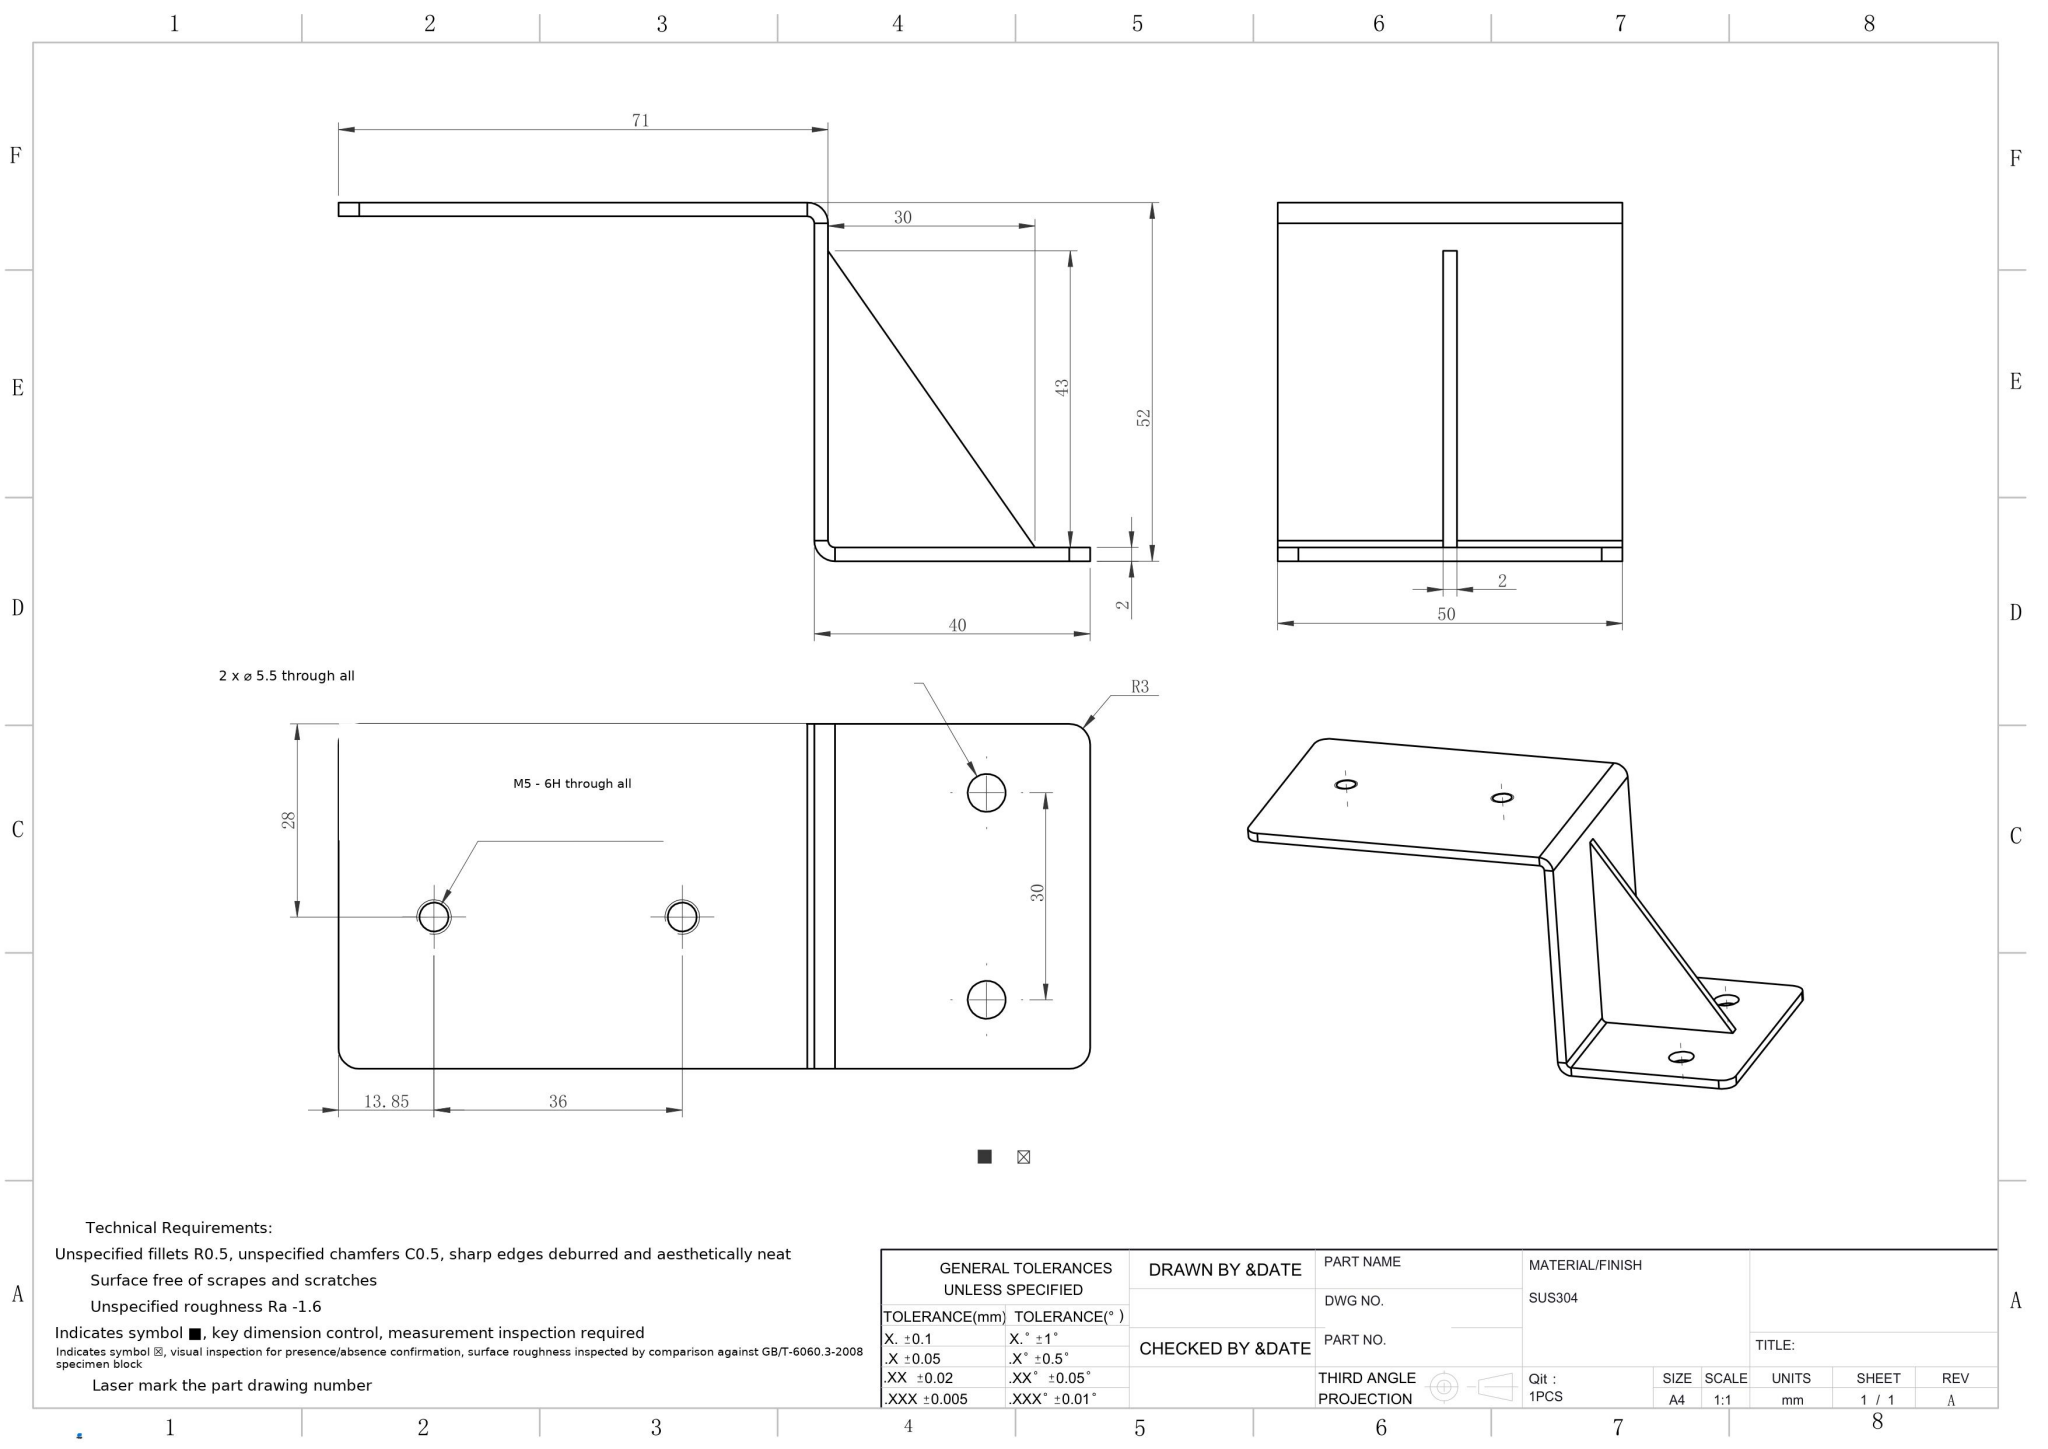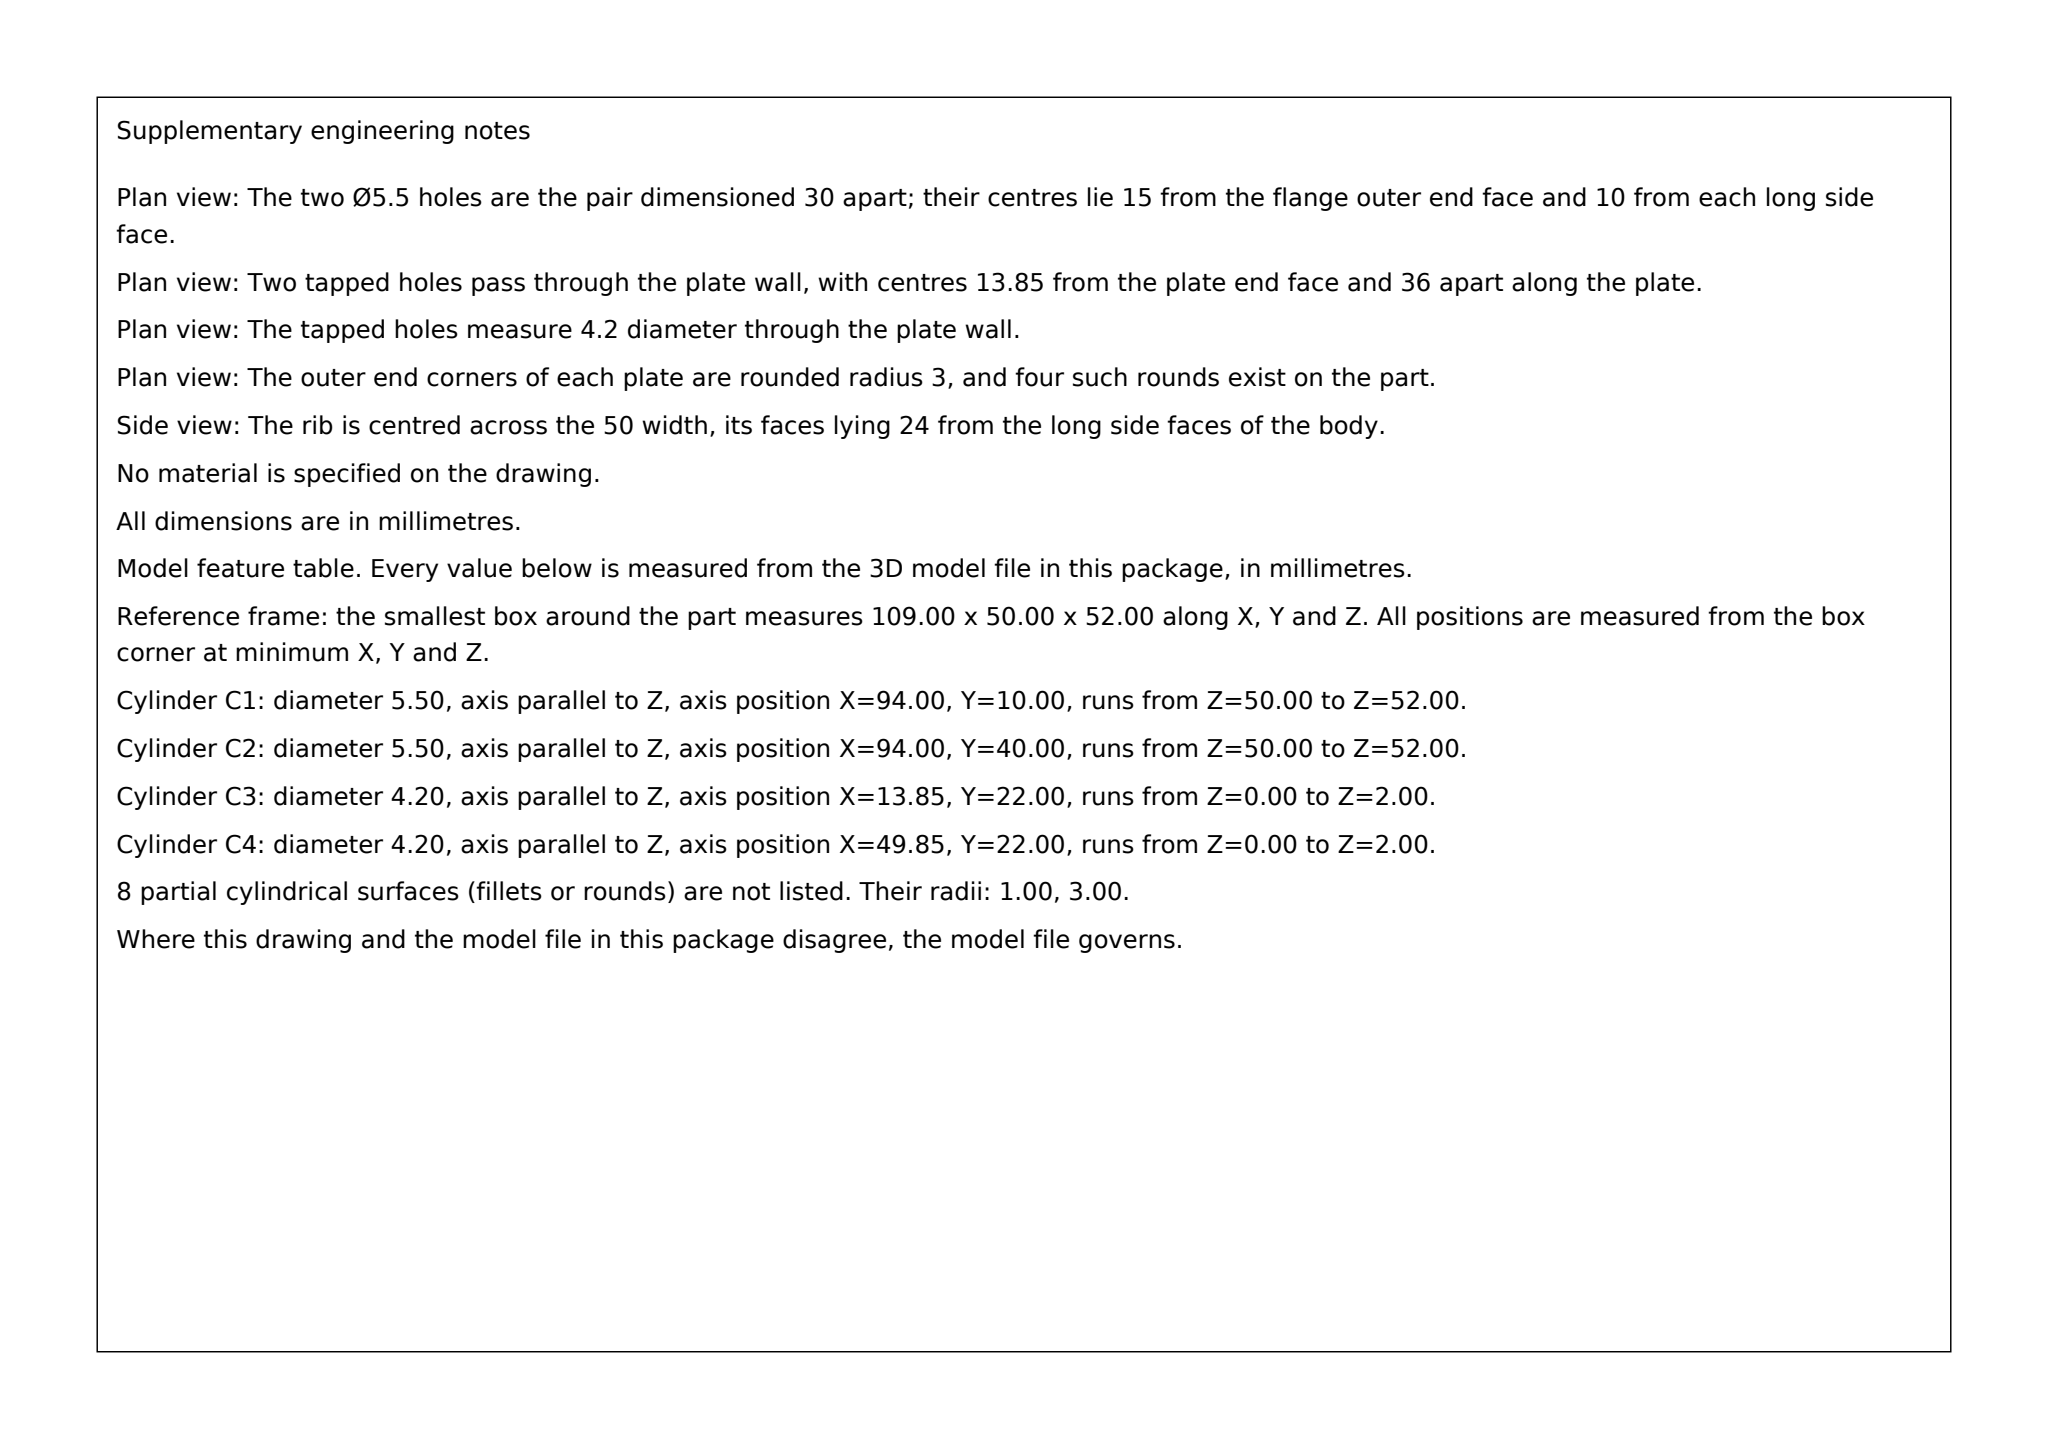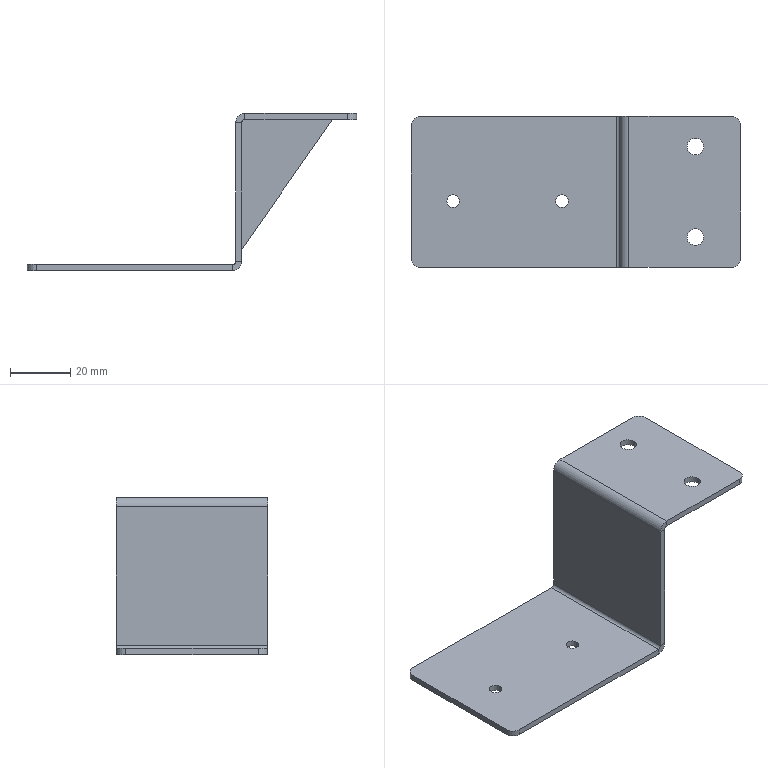Part | SolidWorks | mm | 1 solid | 38 faces | box 109 x 50 x 52 mm | volume 16852 mm3 | plane 21 | cylinder 17 | commonest cylinder face diameters 6 x6 5.5 x4 4.2 x4 2 x3
Drawing notes:
BOTTOM FLANGE: 2X Ø5.5 THRU (2 THK), hole centres 15 from the flange end edge and 10 / 40 from the 50-wide side face (i.e. 30 apart, symmetric about the width centreline). | from the solid: cylinders dia 5.5 axis z at (x=94, y=10) and (x=94, y=40), length 2; bbox_xyz x=109, y=50
2X 90° BEND: INSIDE RADIUS R1, OUTSIDE RADIUS R3 (2 THK) - overrides the general 'unspecified fillets R0.5' note; bend axes at x=68 and x=72. | from the solid: cylinders dia 2.0 axis y at (68,z=3) and (72,z=49) with concentric dia 6.0 axis y at same positions
TRIANGULAR GUSSET RIB 2 THK CENTRED ON THE 50 WIDTH CENTRELINE: rib faces at 24 and 26 from the datum side face (Y=0). | from the solid: axis_planes normal y at offsets 24.0 and 26.0, with outer faces y=0 and y=50
4X R3 OUTLINE CORNER RADII on the flange outline; radii centres 3 from each adjacent edge. | from the solid: cylinders dia 6.0 axis z at (3,3), (3,47), (106,3), (106,47), length 2
2X Ø4.2 THRU (2 THK) TAPPED M5-6H THRU ALL; hole centres at Y=22 from the datum side face (Y=0), at X=13.85 and X=49.85 from the flange end edge (X=0). | from the solid: cylinders[dia,axis,pos]: [4.2,"z",[13.85,22.0],len 2.0] and [4.2,"z",[49.85,22.0],len 2.0]
2X Ø5.5 THRU (2 THK) in bottom flange; hole centres at X=94 (15 from the flange end edge at X=109) and Y=10 / Y=40 from the datum side face (Y=0), 30 apart. | from the solid: cylinders[dia,axis,pos]: [5.5,"z",[94.0,10.0],len 2.0] and [5.5,"z",[94.0,40.0],len 2.0]; bbox_xyz x=109
4X R3 outline corner radii on the flange outline; radii centres at (X3,Y3), (X3,Y47), (X106,Y3) and (X106,Y47) from the datum corner. | from the solid: cylinders[dia,axis,pos]: [6.0,"z",[3.0,3.0]], [6.0,"z",[3.0,47.0]], [6.0,"z",[106.0,3.0]], [6.0,"z",[106.0,47.0]], each len 2.0
2X Ø4.2 THRU (2 THK), TAPPED M5-6H THRU ALL; hole centres Y=22 from datum side face, at X=13.85 and X=49.85 from flange end edge (X=0). | from the solid: cylinders dia 4.2 axis z at (13.85,22) and (49.85,22), length 2
2X Ø5.5 THRU (2 THK) in bottom flange; hole centres X=94 (15 from flange end edge at X=109), Y=10 and Y=40 from datum side face (Y=0), 30 apart. | from the solid: cylinders dia 5.5 axis z at (94,10) and (94,40), length 2
4X R3 outline corner radii on flange outline; radii centres (X3,Y3), (X3,Y47), (X106,Y3), (X106,Y47) from datum corner. | from the solid: cylinders dia 6.0 axis z at (3,3), (3,47), (106,3), (106,47), length 2